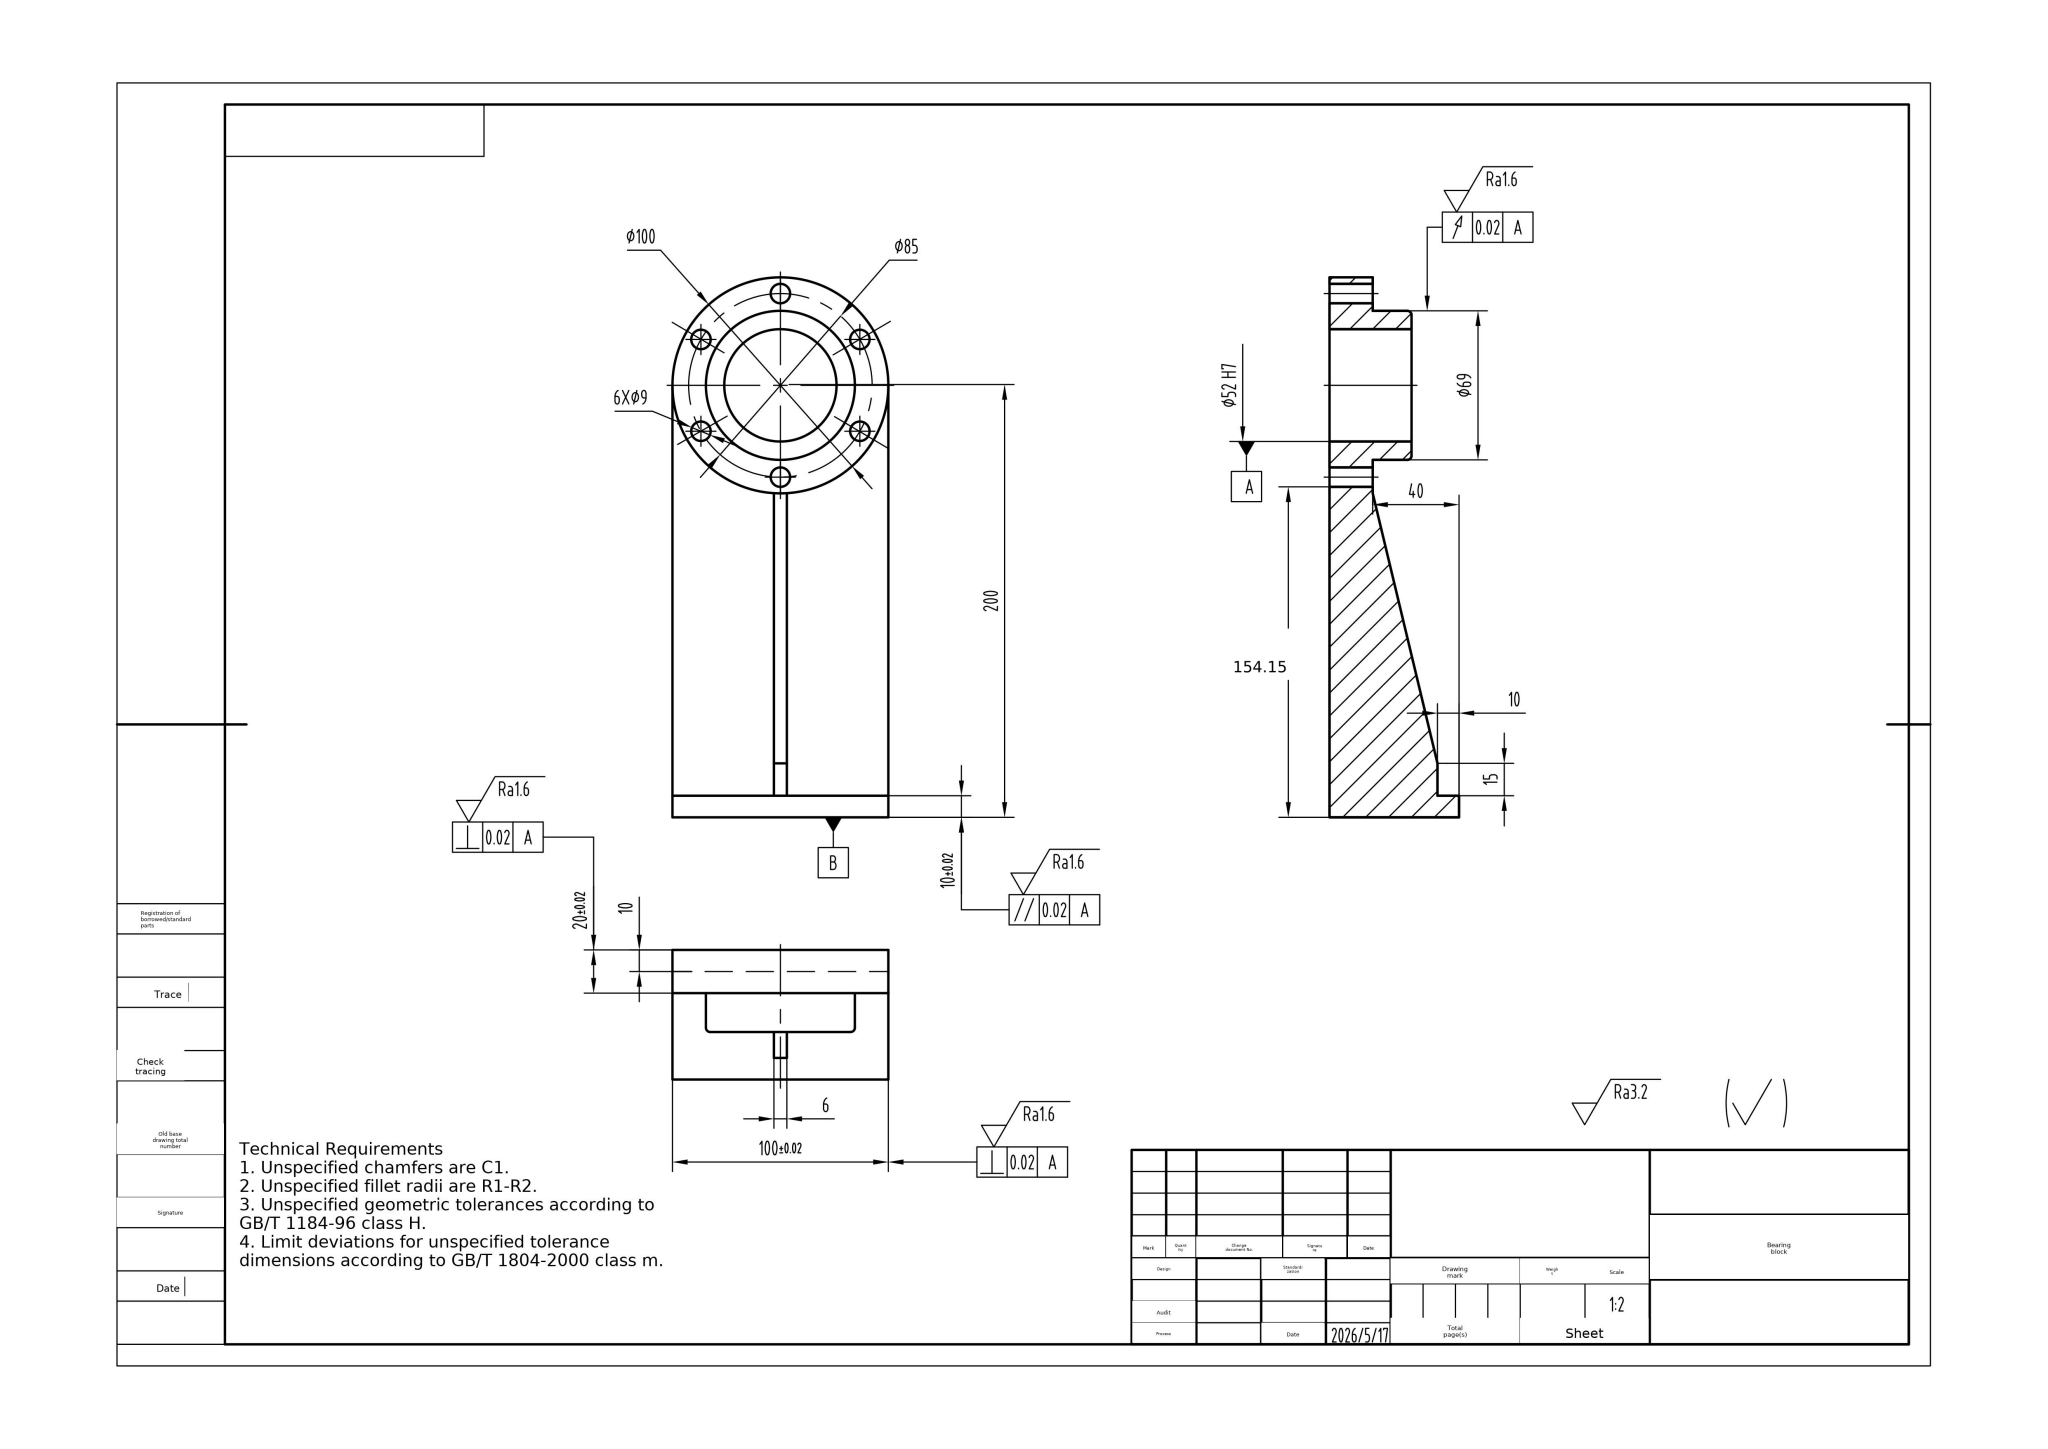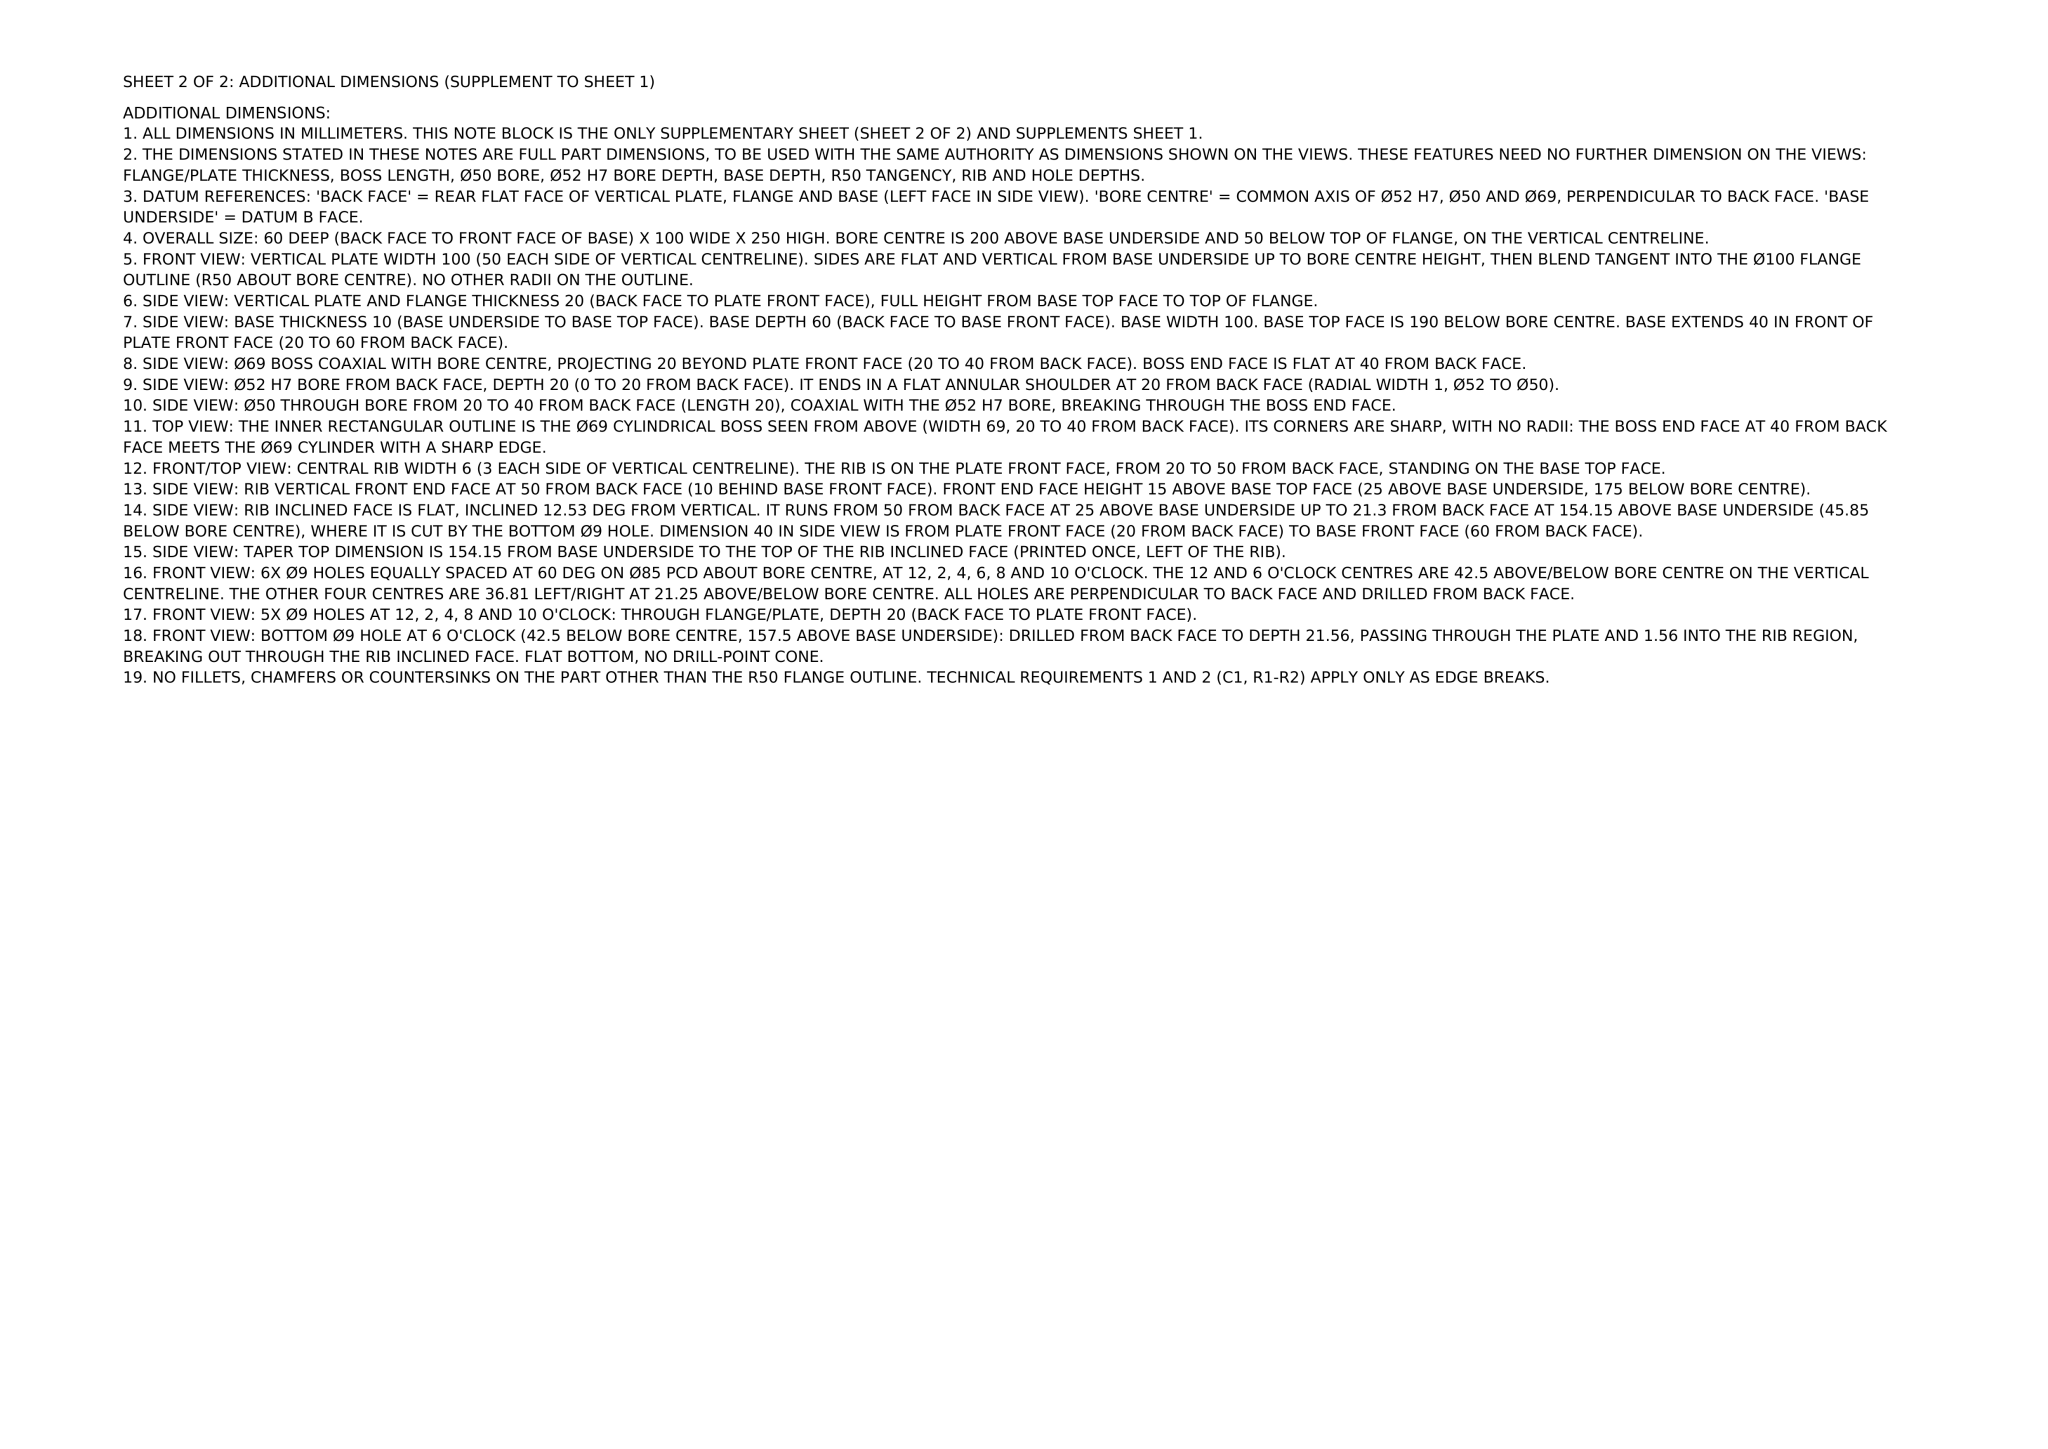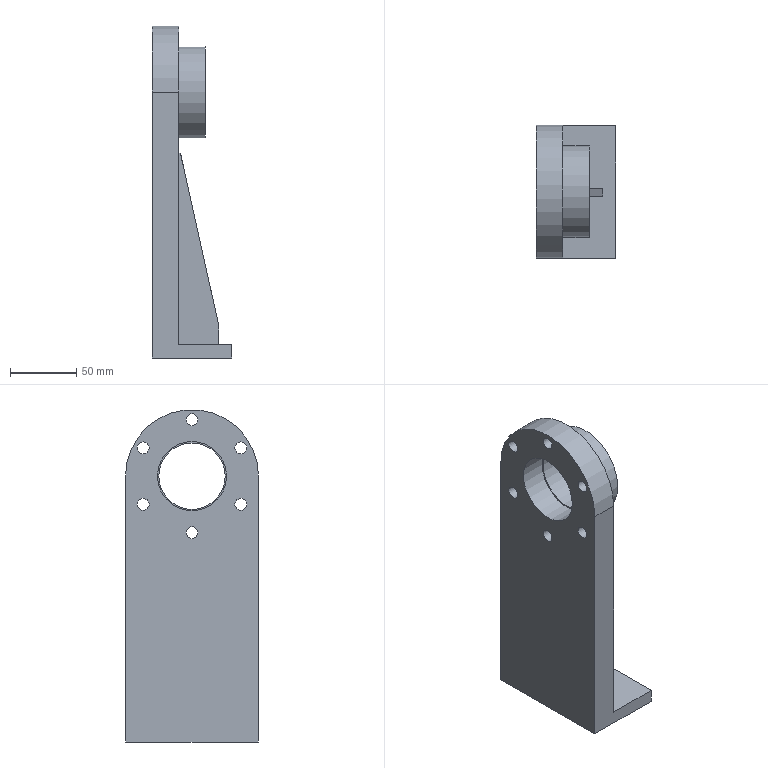Part | NX | mm | 1 solid | 23 faces | box 60 x 100 x 250 mm | volume 518768 mm3 | plane 13 | cylinder 10 | commonest cylinder face diameters 9 x6 100 x1 52 x1 69 x1 50 x1
STEP:
#1=CARTESIAN_POINT('',(0.,0.,0.));
#2=DIRECTION('',(0.,0.,1.));
#3=DIRECTION('',(1.,0.,0.));
#4=AXIS2_PLACEMENT_3D('',#1,#2,#3);
#5=(LENGTH_UNIT()NAMED_UNIT(*)SI_UNIT(.MILLI.,.METRE.));
#6=UNCERTAINTY_MEASURE_WITH_UNIT(LENGTH_MEASURE(0.00002),#5,'','');
#7=(NAMED_UNIT(*)PLANE_ANGLE_UNIT()SI_UNIT($,.RADIAN.));
#8=PLANE_ANGLE_MEASURE_WITH_UNIT(PLANE_ANGLE_MEASURE(0.01745),#7);
#9=DIMENSIONAL_EXPONENTS(0.,0.,0.,0.,0.,0.,0.);
#10=(CONVERSION_BASED_UNIT('',#8)NAMED_UNIT(#9)PLANE_ANGLE_UNIT());
#11=(NAMED_UNIT(*)SI_UNIT($,.STERADIAN.)SOLID_ANGLE_UNIT());
#12=(GEOMETRIC_REPRESENTATION_CONTEXT(3)GLOBAL_UNCERTAINTY_ASSIGNED_CONTEXT((#6))GLOBAL_UNIT_ASSIGNED_CONTEXT((#5,#10,#11))REPRESENTATION_CONTEXT('',''));
#13=SHAPE_REPRESENTATION('',(#4),#12);
#14=CARTESIAN_POINT('',(20.,-36.806,16.75));
#15=VERTEX_POINT('',#14);
#16=CARTESIAN_POINT('',(20.,-36.806,21.25));
#17=DIRECTION('',(1.,0.,0.));
#18=DIRECTION('',(0.,0.,-1.));
#19=AXIS2_PLACEMENT_3D('',#16,#17,#18);
#20=CIRCLE('',#19,4.5);
#21=EDGE_CURVE('',#15,#15,#20,.T.);
#22=ORIENTED_EDGE('',*,*,#21,.F.);
#23=EDGE_LOOP('',(#22));
#24=FACE_BOUND('',#23,.T.);
#25=CARTESIAN_POINT('',(20.,3.,-45.854));
#26=VERTEX_POINT('',#25);
#27=CARTESIAN_POINT('',(20.,-3.,-45.854));
#28=VERTEX_POINT('',#27);
#29=CARTESIAN_POINT('',(20.,0.,-42.5));
#30=DIRECTION('',(1.,0.,0.));
#31=DIRECTION('',(0.,0.,-1.));
#32=AXIS2_PLACEMENT_3D('',#29,#30,#31);
#33=CIRCLE('',#32,4.5);
#34=EDGE_CURVE('',#26,#28,#33,.T.);
#35=ORIENTED_EDGE('',*,*,#34,.F.);
#36=CARTESIAN_POINT('',(20.,3.,-190.));
#37=VERTEX_POINT('',#36);
#38=CARTESIAN_POINT('',(20.,3.,-40.));
#39=DIRECTION('',(0.,0.,-1.));
#40=VECTOR('',#39,1.);
#41=LINE('',#38,#40);
#42=EDGE_CURVE('',#26,#37,#41,.T.);
#43=ORIENTED_EDGE('',*,*,#42,.T.);
#44=CARTESIAN_POINT('',(20.,50.,-190.));
#45=VERTEX_POINT('',#44);
#46=CARTESIAN_POINT('',(20.,0.,-190.));
#47=DIRECTION('',(0.,1.,0.));
#48=VECTOR('',#47,1.);
#49=LINE('',#46,#48);
#50=EDGE_CURVE('',#37,#45,#49,.T.);
#51=ORIENTED_EDGE('',*,*,#50,.T.);
#52=CARTESIAN_POINT('',(20.,50.,0.));
#53=VERTEX_POINT('',#52);
#54=CARTESIAN_POINT('',(20.,50.,-200.));
#55=DIRECTION('',(0.,0.,1.));
#56=VECTOR('',#55,1.);
#57=LINE('',#54,#56);
#58=EDGE_CURVE('',#45,#53,#57,.T.);
#59=ORIENTED_EDGE('',*,*,#58,.T.);
#60=CARTESIAN_POINT('',(20.,-50.,0.));
#61=VERTEX_POINT('',#60);
#62=CARTESIAN_POINT('',(20.,0.,0.));
#63=DIRECTION('',(1.,0.,0.));
#64=DIRECTION('',(0.,1.,-0.));
#65=AXIS2_PLACEMENT_3D('',#62,#63,#64);
#66=CIRCLE('',#65,50.);
#67=EDGE_CURVE('',#53,#61,#66,.T.);
#68=ORIENTED_EDGE('',*,*,#67,.T.);
#69=CARTESIAN_POINT('',(20.,-50.,-190.));
#70=VERTEX_POINT('',#69);
#71=CARTESIAN_POINT('',(20.,-50.,0.));
#72=DIRECTION('',(0.,0.,-1.));
#73=VECTOR('',#72,1.);
#74=LINE('',#71,#73);
#75=EDGE_CURVE('',#61,#70,#74,.T.);
#76=ORIENTED_EDGE('',*,*,#75,.T.);
#77=CARTESIAN_POINT('',(20.,-3.,-190.));
#78=VERTEX_POINT('',#77);
#79=CARTESIAN_POINT('',(20.,0.,-190.));
#80=DIRECTION('',(0.,1.,0.));
#81=VECTOR('',#80,1.);
#82=LINE('',#79,#81);
#83=EDGE_CURVE('',#70,#78,#82,.T.);
#84=ORIENTED_EDGE('',*,*,#83,.T.);
#85=CARTESIAN_POINT('',(20.,-3.,-40.));
#86=DIRECTION('',(0.,0.,-1.));
#87=VECTOR('',#86,1.);
#88=LINE('',#85,#87);
#89=EDGE_CURVE('',#28,#78,#88,.T.);
#90=ORIENTED_EDGE('',*,*,#89,.F.);
#91=EDGE_LOOP('',(#35,#43,#51,#59,#68,#76,#84,#90));
#92=FACE_BOUND('',#91,.T.);
#93=CARTESIAN_POINT('',(20.,0.,38.));
#94=VERTEX_POINT('',#93);
#95=CARTESIAN_POINT('',(20.,0.,42.5));
#96=DIRECTION('',(1.,0.,0.));
#97=DIRECTION('',(0.,0.,-1.));
#98=AXIS2_PLACEMENT_3D('',#95,#96,#97);
#99=CIRCLE('',#98,4.5);
#100=EDGE_CURVE('',#94,#94,#99,.T.);
#101=ORIENTED_EDGE('',*,*,#100,.F.);
#102=EDGE_LOOP('',(#101));
#103=FACE_BOUND('',#102,.T.);
#104=CARTESIAN_POINT('',(20.,36.806,-25.75));
#105=VERTEX_POINT('',#104);
#106=CARTESIAN_POINT('',(20.,36.806,-21.25));
#107=DIRECTION('',(1.,0.,0.));
#108=DIRECTION('',(0.,0.,-1.));
#109=AXIS2_PLACEMENT_3D('',#106,#107,#108);
#110=CIRCLE('',#109,4.5);
#111=EDGE_CURVE('',#105,#105,#110,.T.);
#112=ORIENTED_EDGE('',*,*,#111,.F.);
#113=EDGE_LOOP('',(#112));
#114=FACE_BOUND('',#113,.T.);
#115=CARTESIAN_POINT('',(20.,-36.806,-25.75));
#116=VERTEX_POINT('',#115);
#117=CARTESIAN_POINT('',(20.,-36.806,-21.25));
#118=DIRECTION('',(1.,0.,0.));
#119=DIRECTION('',(0.,0.,-1.));
#120=AXIS2_PLACEMENT_3D('',#117,#118,#119);
#121=CIRCLE('',#120,4.5);
#122=EDGE_CURVE('',#116,#116,#121,.T.);
#123=ORIENTED_EDGE('',*,*,#122,.F.);
#124=EDGE_LOOP('',(#123));
#125=FACE_BOUND('',#124,.T.);
#126=CARTESIAN_POINT('',(20.,36.806,16.75));
#127=VERTEX_POINT('',#126);
#128=CARTESIAN_POINT('',(20.,36.806,21.25));
#129=DIRECTION('',(1.,0.,0.));
#130=DIRECTION('',(0.,0.,-1.));
#131=AXIS2_PLACEMENT_3D('',#128,#129,#130);
#132=CIRCLE('',#131,4.5);
#133=EDGE_CURVE('',#127,#127,#132,.T.);
#134=ORIENTED_EDGE('',*,*,#133,.F.);
#135=EDGE_LOOP('',(#134));
#136=FACE_BOUND('',#135,.T.);
#137=CARTESIAN_POINT('',(20.,34.5,-0.));
#138=VERTEX_POINT('',#137);
#139=CARTESIAN_POINT('',(20.,0.,0.));
#140=DIRECTION('',(1.,0.,0.));
#141=DIRECTION('',(0.,1.,-0.));
#142=AXIS2_PLACEMENT_3D('',#139,#140,#141);
#143=CIRCLE('',#142,34.5);
#144=EDGE_CURVE('',#138,#138,#143,.T.);
#145=ORIENTED_EDGE('',*,*,#144,.F.);
#146=EDGE_LOOP('',(#145));
#147=FACE_BOUND('',#146,.T.);
#148=CARTESIAN_POINT('',(20.,0.,0.));
#149=DIRECTION('',(1.,0.,0.));
#150=DIRECTION('',(0.,0.,-1.));
#151=AXIS2_PLACEMENT_3D('',#148,#149,#150);
#152=PLANE('',#151);
#153=ADVANCED_FACE('',(#24,#92,#103,#114,#125,#136,#147),#152,.T.);
#154=CARTESIAN_POINT('',(60.,-50.,-200.));
#155=VERTEX_POINT('',#154);
#156=CARTESIAN_POINT('',(0.,-50.,-200.));
#157=VERTEX_POINT('',#156);
#158=CARTESIAN_POINT('',(20.,-50.,-200.));
#159=DIRECTION('',(-1.,0.,0.));
#160=VECTOR('',#159,1.);
#161=LINE('',#158,#160);
#162=EDGE_CURVE('',#155,#157,#161,.T.);
#163=ORIENTED_EDGE('',*,*,#162,.F.);
#164=CARTESIAN_POINT('',(60.,-50.,-190.));
#165=VERTEX_POINT('',#164);
#166=CARTESIAN_POINT('',(60.,-50.,-190.));
#167=DIRECTION('',(0.,0.,-1.));
#168=VECTOR('',#167,1.);
#169=LINE('',#166,#168);
#170=EDGE_CURVE('',#165,#155,#169,.T.);
#171=ORIENTED_EDGE('',*,*,#170,.F.);
#172=CARTESIAN_POINT('',(60.,-50.,-190.));
#173=DIRECTION('',(-1.,0.,0.));
#174=VECTOR('',#173,1.);
#175=LINE('',#172,#174);
#176=EDGE_CURVE('',#165,#70,#175,.T.);
#177=ORIENTED_EDGE('',*,*,#176,.T.);
#178=ORIENTED_EDGE('',*,*,#75,.F.);
#179=CARTESIAN_POINT('',(0.,-50.,0.));
#180=VERTEX_POINT('',#179);
#181=CARTESIAN_POINT('',(20.,-50.,0.));
#182=DIRECTION('',(-1.,0.,0.));
#183=VECTOR('',#182,1.);
#184=LINE('',#181,#183);
#185=EDGE_CURVE('',#61,#180,#184,.T.);
#186=ORIENTED_EDGE('',*,*,#185,.T.);
#187=CARTESIAN_POINT('',(0.,-50.,0.));
#188=DIRECTION('',(0.,0.,-1.));
#189=VECTOR('',#188,1.);
#190=LINE('',#187,#189);
#191=EDGE_CURVE('',#180,#157,#190,.T.);
#192=ORIENTED_EDGE('',*,*,#191,.T.);
#193=EDGE_LOOP('',(#163,#171,#177,#178,#186,#192));
#194=FACE_OUTER_BOUND('',#193,.T.);
#195=CARTESIAN_POINT('',(20.,-50.,0.));
#196=DIRECTION('',(0.,1.,0.));
#197=DIRECTION('',(0.,-0.,1.));
#198=AXIS2_PLACEMENT_3D('',#195,#196,#197);
#199=PLANE('',#198);
#200=ADVANCED_FACE('',(#194),#199,.F.);
#201=CARTESIAN_POINT('',(0.,50.,-200.));
#202=VERTEX_POINT('',#201);
#203=CARTESIAN_POINT('',(0.,-50.,-200.));
#204=DIRECTION('',(0.,1.,0.));
#205=VECTOR('',#204,1.);
#206=LINE('',#203,#205);
#207=EDGE_CURVE('',#157,#202,#206,.T.);
#208=ORIENTED_EDGE('',*,*,#207,.T.);
#209=CARTESIAN_POINT('',(60.,50.,-200.));
#210=VERTEX_POINT('',#209);
#211=CARTESIAN_POINT('',(20.,50.,-200.));
#212=DIRECTION('',(-1.,0.,0.));
#213=VECTOR('',#212,1.);
#214=LINE('',#211,#213);
#215=EDGE_CURVE('',#210,#202,#214,.T.);
#216=ORIENTED_EDGE('',*,*,#215,.F.);
#217=CARTESIAN_POINT('',(60.,50.,-200.));
#218=DIRECTION('',(-0.,-1.,0.));
#219=VECTOR('',#218,1.);
#220=LINE('',#217,#219);
#221=EDGE_CURVE('',#210,#155,#220,.T.);
#222=ORIENTED_EDGE('',*,*,#221,.T.);
#223=ORIENTED_EDGE('',*,*,#162,.T.);
#224=EDGE_LOOP('',(#208,#216,#222,#223));
#225=FACE_OUTER_BOUND('',#224,.T.);
#226=CARTESIAN_POINT('',(20.,-50.,-200.));
#227=DIRECTION('',(0.,0.,1.));
#228=DIRECTION('',(1.,0.,0.));
#229=AXIS2_PLACEMENT_3D('',#226,#227,#228);
#230=PLANE('',#229);
#231=ADVANCED_FACE('',(#225),#230,.F.);
#232=CARTESIAN_POINT('',(0.,50.,0.));
#233=VERTEX_POINT('',#232);
#234=CARTESIAN_POINT('',(0.,50.,-200.));
#235=DIRECTION('',(0.,0.,1.));
#236=VECTOR('',#235,1.);
#237=LINE('',#234,#236);
#238=EDGE_CURVE('',#202,#233,#237,.T.);
#239=ORIENTED_EDGE('',*,*,#238,.T.);
#240=CARTESIAN_POINT('',(20.,50.,0.));
#241=DIRECTION('',(-1.,0.,0.));
#242=VECTOR('',#241,1.);
#243=LINE('',#240,#242);
#244=EDGE_CURVE('',#53,#233,#243,.T.);
#245=ORIENTED_EDGE('',*,*,#244,.F.);
#246=ORIENTED_EDGE('',*,*,#58,.F.);
#247=CARTESIAN_POINT('',(60.,50.,-190.));
#248=VERTEX_POINT('',#247);
#249=CARTESIAN_POINT('',(0.,50.,-190.));
#250=DIRECTION('',(1.,-0.,0.));
#251=VECTOR('',#250,1.);
#252=LINE('',#249,#251);
#253=EDGE_CURVE('',#45,#248,#252,.T.);
#254=ORIENTED_EDGE('',*,*,#253,.T.);
#255=CARTESIAN_POINT('',(60.,50.,-190.));
#256=DIRECTION('',(0.,0.,-1.));
#257=VECTOR('',#256,1.);
#258=LINE('',#255,#257);
#259=EDGE_CURVE('',#248,#210,#258,.T.);
#260=ORIENTED_EDGE('',*,*,#259,.T.);
#261=ORIENTED_EDGE('',*,*,#215,.T.);
#262=EDGE_LOOP('',(#239,#245,#246,#254,#260,#261));
#263=FACE_OUTER_BOUND('',#262,.T.);
#264=CARTESIAN_POINT('',(20.,50.,-200.));
#265=DIRECTION('',(0.,-1.,0.));
#266=DIRECTION('',(0.,0.,-1.));
#267=AXIS2_PLACEMENT_3D('',#264,#265,#266);
#268=PLANE('',#267);
#269=ADVANCED_FACE('',(#263),#268,.F.);
#270=CARTESIAN_POINT('',(0.,0.,0.));
#271=DIRECTION('',(1.,0.,0.));
#272=DIRECTION('',(0.,1.,-0.));
#273=AXIS2_PLACEMENT_3D('',#270,#271,#272);
#274=CIRCLE('',#273,50.);
#275=EDGE_CURVE('',#233,#180,#274,.T.);
#276=ORIENTED_EDGE('',*,*,#275,.T.);
#277=ORIENTED_EDGE('',*,*,#185,.F.);
#278=ORIENTED_EDGE('',*,*,#67,.F.);
#279=ORIENTED_EDGE('',*,*,#244,.T.);
#280=EDGE_LOOP('',(#276,#277,#278,#279));
#281=FACE_OUTER_BOUND('',#280,.T.);
#282=CARTESIAN_POINT('',(20.,0.,0.));
#283=DIRECTION('',(-1.,0.,0.));
#284=DIRECTION('',(0.,0.,1.));
#285=AXIS2_PLACEMENT_3D('',#282,#283,#284);
#286=CYLINDRICAL_SURFACE('',#285,50.);
#287=ADVANCED_FACE('',(#281),#286,.T.);
#288=CARTESIAN_POINT('',(20.,26.,-0.));
#289=VERTEX_POINT('',#288);
#290=CARTESIAN_POINT('',(20.,0.,0.));
#291=DIRECTION('',(1.,0.,0.));
#292=DIRECTION('',(0.,1.,-0.));
#293=AXIS2_PLACEMENT_3D('',#290,#291,#292);
#294=CIRCLE('',#293,26.);
#295=EDGE_CURVE('',#289,#289,#294,.T.);
#296=ORIENTED_EDGE('',*,*,#295,.T.);
#297=EDGE_LOOP('',(#296));
#298=FACE_BOUND('',#297,.T.);
#299=CARTESIAN_POINT('',(0.,26.,-0.));
#300=VERTEX_POINT('',#299);
#301=CARTESIAN_POINT('',(0.,0.,0.));
#302=DIRECTION('',(1.,0.,0.));
#303=DIRECTION('',(0.,1.,-0.));
#304=AXIS2_PLACEMENT_3D('',#301,#302,#303);
#305=CIRCLE('',#304,26.);
#306=EDGE_CURVE('',#300,#300,#305,.T.);
#307=ORIENTED_EDGE('',*,*,#306,.F.);
#308=EDGE_LOOP('',(#307));
#309=FACE_BOUND('',#308,.T.);
#310=CARTESIAN_POINT('',(20.,0.,0.));
#311=DIRECTION('',(-1.,0.,0.));
#312=DIRECTION('',(0.,0.,1.));
#313=AXIS2_PLACEMENT_3D('',#310,#311,#312);
#314=CYLINDRICAL_SURFACE('',#313,26.);
#315=ADVANCED_FACE('',(#298,#309),#314,.F.);
#316=CARTESIAN_POINT('',(0.,-36.806,16.75));
#317=VERTEX_POINT('',#316);
#318=CARTESIAN_POINT('',(0.,-36.806,21.25));
#319=DIRECTION('',(1.,0.,0.));
#320=DIRECTION('',(0.,0.,-1.));
#321=AXIS2_PLACEMENT_3D('',#318,#319,#320);
#322=CIRCLE('',#321,4.5);
#323=EDGE_CURVE('',#317,#317,#322,.T.);
#324=ORIENTED_EDGE('',*,*,#323,.T.);
#325=EDGE_LOOP('',(#324));
#326=FACE_BOUND('',#325,.T.);
#327=CARTESIAN_POINT('',(0.,0.,-47.));
#328=VERTEX_POINT('',#327);
#329=CARTESIAN_POINT('',(0.,0.,-42.5));
#330=DIRECTION('',(1.,0.,0.));
#331=DIRECTION('',(0.,0.,-1.));
#332=AXIS2_PLACEMENT_3D('',#329,#330,#331);
#333=CIRCLE('',#332,4.5);
#334=EDGE_CURVE('',#328,#328,#333,.T.);
#335=ORIENTED_EDGE('',*,*,#334,.T.);
#336=EDGE_LOOP('',(#335));
#337=FACE_BOUND('',#336,.T.);
#338=CARTESIAN_POINT('',(0.,0.,38.));
#339=VERTEX_POINT('',#338);
#340=CARTESIAN_POINT('',(0.,0.,42.5));
#341=DIRECTION('',(1.,0.,0.));
#342=DIRECTION('',(0.,0.,-1.));
#343=AXIS2_PLACEMENT_3D('',#340,#341,#342);
#344=CIRCLE('',#343,4.5);
#345=EDGE_CURVE('',#339,#339,#344,.T.);
#346=ORIENTED_EDGE('',*,*,#345,.T.);
#347=EDGE_LOOP('',(#346));
#348=FACE_BOUND('',#347,.T.);
#349=CARTESIAN_POINT('',(0.,36.806,-25.75));
#350=VERTEX_POINT('',#349);
#351=CARTESIAN_POINT('',(0.,36.806,-21.25));
#352=DIRECTION('',(1.,0.,0.));
#353=DIRECTION('',(0.,0.,-1.));
#354=AXIS2_PLACEMENT_3D('',#351,#352,#353);
#355=CIRCLE('',#354,4.5);
#356=EDGE_CURVE('',#350,#350,#355,.T.);
#357=ORIENTED_EDGE('',*,*,#356,.T.);
#358=EDGE_LOOP('',(#357));
#359=FACE_BOUND('',#358,.T.);
#360=CARTESIAN_POINT('',(0.,-36.806,-25.75));
#361=VERTEX_POINT('',#360);
#362=CARTESIAN_POINT('',(0.,-36.806,-21.25));
#363=DIRECTION('',(1.,0.,0.));
#364=DIRECTION('',(0.,0.,-1.));
#365=AXIS2_PLACEMENT_3D('',#362,#363,#364);
#366=CIRCLE('',#365,4.5);
#367=EDGE_CURVE('',#361,#361,#366,.T.);
#368=ORIENTED_EDGE('',*,*,#367,.T.);
#369=EDGE_LOOP('',(#368));
#370=FACE_BOUND('',#369,.T.);
#371=CARTESIAN_POINT('',(0.,36.806,16.75));
#372=VERTEX_POINT('',#371);
#373=CARTESIAN_POINT('',(0.,36.806,21.25));
#374=DIRECTION('',(1.,0.,0.));
#375=DIRECTION('',(0.,0.,-1.));
#376=AXIS2_PLACEMENT_3D('',#373,#374,#375);
#377=CIRCLE('',#376,4.5);
#378=EDGE_CURVE('',#372,#372,#377,.T.);
#379=ORIENTED_EDGE('',*,*,#378,.T.);
#380=EDGE_LOOP('',(#379));
#381=FACE_BOUND('',#380,.T.);
#382=ORIENTED_EDGE('',*,*,#207,.F.);
#383=ORIENTED_EDGE('',*,*,#191,.F.);
#384=ORIENTED_EDGE('',*,*,#275,.F.);
#385=ORIENTED_EDGE('',*,*,#238,.F.);
#386=EDGE_LOOP('',(#382,#383,#384,#385));
#387=FACE_BOUND('',#386,.T.);
#388=ORIENTED_EDGE('',*,*,#306,.T.);
#389=EDGE_LOOP('',(#388));
#390=FACE_BOUND('',#389,.T.);
#391=CARTESIAN_POINT('',(0.,0.,0.));
#392=DIRECTION('',(1.,0.,0.));
#393=DIRECTION('',(0.,0.,-1.));
#394=AXIS2_PLACEMENT_3D('',#391,#392,#393);
#395=PLANE('',#394);
#396=ADVANCED_FACE('',(#326,#337,#348,#359,#370,#381,#387,#390),#395,.F.);
#397=CARTESIAN_POINT('',(40.,34.5,-0.));
#398=VERTEX_POINT('',#397);
#399=CARTESIAN_POINT('',(40.,0.,0.));
#400=DIRECTION('',(1.,0.,0.));
#401=DIRECTION('',(0.,1.,-0.));
#402=AXIS2_PLACEMENT_3D('',#399,#400,#401);
#403=CIRCLE('',#402,34.5);
#404=EDGE_CURVE('',#398,#398,#403,.T.);
#405=ORIENTED_EDGE('',*,*,#404,.F.);
#406=EDGE_LOOP('',(#405));
#407=FACE_BOUND('',#406,.T.);
#408=ORIENTED_EDGE('',*,*,#144,.T.);
#409=EDGE_LOOP('',(#408));
#410=FACE_BOUND('',#409,.T.);
#411=CARTESIAN_POINT('',(40.,0.,0.));
#412=DIRECTION('',(-1.,0.,0.));
#413=DIRECTION('',(0.,0.,1.));
#414=AXIS2_PLACEMENT_3D('',#411,#412,#413);
#415=CYLINDRICAL_SURFACE('',#414,34.5);
#416=ADVANCED_FACE('',(#407,#410),#415,.T.);
#417=CARTESIAN_POINT('',(40.,25.,-0.));
#418=VERTEX_POINT('',#417);
#419=CARTESIAN_POINT('',(40.,0.,0.));
#420=DIRECTION('',(1.,0.,0.));
#421=DIRECTION('',(0.,1.,-0.));
#422=AXIS2_PLACEMENT_3D('',#419,#420,#421);
#423=CIRCLE('',#422,25.);
#424=EDGE_CURVE('',#418,#418,#423,.T.);
#425=ORIENTED_EDGE('',*,*,#424,.T.);
#426=EDGE_LOOP('',(#425));
#427=FACE_BOUND('',#426,.T.);
#428=CARTESIAN_POINT('',(20.,25.,-0.));
#429=VERTEX_POINT('',#428);
#430=CARTESIAN_POINT('',(20.,0.,0.));
#431=DIRECTION('',(1.,0.,0.));
#432=DIRECTION('',(0.,1.,-0.));
#433=AXIS2_PLACEMENT_3D('',#430,#431,#432);
#434=CIRCLE('',#433,25.);
#435=EDGE_CURVE('',#429,#429,#434,.T.);
#436=ORIENTED_EDGE('',*,*,#435,.F.);
#437=EDGE_LOOP('',(#436));
#438=FACE_BOUND('',#437,.T.);
#439=CARTESIAN_POINT('',(40.,0.,0.));
#440=DIRECTION('',(-1.,0.,0.));
#441=DIRECTION('',(0.,0.,1.));
#442=AXIS2_PLACEMENT_3D('',#439,#440,#441);
#443=CYLINDRICAL_SURFACE('',#442,25.);
#444=ADVANCED_FACE('',(#427,#438),#443,.F.);
#445=ORIENTED_EDGE('',*,*,#404,.T.);
#446=EDGE_LOOP('',(#445));
#447=FACE_BOUND('',#446,.T.);
#448=ORIENTED_EDGE('',*,*,#424,.F.);
#449=EDGE_LOOP('',(#448));
#450=FACE_BOUND('',#449,.T.);
#451=CARTESIAN_POINT('',(40.,0.,0.));
#452=DIRECTION('',(1.,0.,0.));
#453=DIRECTION('',(0.,0.,-1.));
#454=AXIS2_PLACEMENT_3D('',#451,#452,#453);
#455=PLANE('',#454);
#456=ADVANCED_FACE('',(#447,#450),#455,.T.);
#457=ORIENTED_EDGE('',*,*,#295,.F.);
#458=EDGE_LOOP('',(#457));
#459=FACE_BOUND('',#458,.T.);
#460=ORIENTED_EDGE('',*,*,#435,.T.);
#461=EDGE_LOOP('',(#460));
#462=FACE_BOUND('',#461,.T.);
#463=CARTESIAN_POINT('',(20.,0.,0.));
#464=DIRECTION('',(1.,0.,0.));
#465=DIRECTION('',(0.,0.,-1.));
#466=AXIS2_PLACEMENT_3D('',#463,#464,#465);
#467=PLANE('',#466);
#468=ADVANCED_FACE('',(#459,#462),#467,.F.);
#469=ORIENTED_EDGE('',*,*,#221,.F.);
#470=ORIENTED_EDGE('',*,*,#259,.F.);
#471=CARTESIAN_POINT('',(60.,50.,-190.));
#472=DIRECTION('',(-0.,-1.,0.));
#473=VECTOR('',#472,1.);
#474=LINE('',#471,#473);
#475=EDGE_CURVE('',#248,#165,#474,.T.);
#476=ORIENTED_EDGE('',*,*,#475,.T.);
#477=ORIENTED_EDGE('',*,*,#170,.T.);
#478=EDGE_LOOP('',(#469,#470,#476,#477));
#479=FACE_OUTER_BOUND('',#478,.T.);
#480=CARTESIAN_POINT('',(60.,50.,-190.));
#481=DIRECTION('',(1.,-0.,0.));
#482=DIRECTION('',(0.,1.,0.));
#483=AXIS2_PLACEMENT_3D('',#480,#481,#482);
#484=PLANE('',#483);
#485=ADVANCED_FACE('',(#479),#484,.T.);
#486=ORIENTED_EDGE('',*,*,#50,.F.);
#487=CARTESIAN_POINT('',(50.,3.,-190.));
#488=VERTEX_POINT('',#487);
#489=CARTESIAN_POINT('',(20.,3.,-190.));
#490=DIRECTION('',(1.,0.,-0.));
#491=VECTOR('',#490,1.);
#492=LINE('',#489,#491);
#493=EDGE_CURVE('',#37,#488,#492,.T.);
#494=ORIENTED_EDGE('',*,*,#493,.T.);
#495=CARTESIAN_POINT('',(50.,-3.,-190.));
#496=VERTEX_POINT('',#495);
#497=CARTESIAN_POINT('',(50.,-3.,-190.));
#498=DIRECTION('',(0.,1.,0.));
#499=VECTOR('',#498,1.);
#500=LINE('',#497,#499);
#501=EDGE_CURVE('',#496,#488,#500,.T.);
#502=ORIENTED_EDGE('',*,*,#501,.F.);
#503=CARTESIAN_POINT('',(20.,-3.,-190.));
#504=DIRECTION('',(1.,0.,-0.));
#505=VECTOR('',#504,1.);
#506=LINE('',#503,#505);
#507=EDGE_CURVE('',#78,#496,#506,.T.);
#508=ORIENTED_EDGE('',*,*,#507,.F.);
#509=ORIENTED_EDGE('',*,*,#83,.F.);
#510=ORIENTED_EDGE('',*,*,#176,.F.);
#511=ORIENTED_EDGE('',*,*,#475,.F.);
#512=ORIENTED_EDGE('',*,*,#253,.F.);
#513=EDGE_LOOP('',(#486,#494,#502,#508,#509,#510,#511,#512));
#514=FACE_OUTER_BOUND('',#513,.T.);
#515=CARTESIAN_POINT('',(0.,0.,-190.));
#516=DIRECTION('',(0.,0.,-1.));
#517=DIRECTION('',(-1.,0.,0.));
#518=AXIS2_PLACEMENT_3D('',#515,#516,#517);
#519=PLANE('',#518);
#520=ADVANCED_FACE('',(#514),#519,.F.);
#521=CARTESIAN_POINT('',(50.,3.,-175.));
#522=VERTEX_POINT('',#521);
#523=CARTESIAN_POINT('',(21.301,3.,-45.854));
#524=VERTEX_POINT('',#523);
#525=CARTESIAN_POINT('',(50.,3.,-175.));
#526=DIRECTION('',(-0.2169,0.,0.9762));
#527=VECTOR('',#526,1.);
#528=LINE('',#525,#527);
#529=EDGE_CURVE('',#522,#524,#528,.T.);
#530=ORIENTED_EDGE('',*,*,#529,.T.);
#531=CARTESIAN_POINT('',(21.301,-3.,-45.854));
#532=VERTEX_POINT('',#531);
#533=CARTESIAN_POINT('',(20.556,0.,-42.5));
#534=DIRECTION('',(-0.9762,0.,-0.2169));
#535=DIRECTION('',(0.2169,0.,-0.9762));
#536=AXIS2_PLACEMENT_3D('',#533,#534,#535);
#537=ELLIPSE('',#536,4.61,4.5);
#538=EDGE_CURVE('',#524,#532,#537,.T.);
#539=ORIENTED_EDGE('',*,*,#538,.T.);
#540=CARTESIAN_POINT('',(50.,-3.,-175.));
#541=VERTEX_POINT('',#540);
#542=CARTESIAN_POINT('',(50.,-3.,-175.));
#543=DIRECTION('',(-0.2169,0.,0.9762));
#544=VECTOR('',#543,1.);
#545=LINE('',#542,#544);
#546=EDGE_CURVE('',#541,#532,#545,.T.);
#547=ORIENTED_EDGE('',*,*,#546,.F.);
#548=CARTESIAN_POINT('',(50.,-3.,-175.));
#549=DIRECTION('',(0.,1.,0.));
#550=VECTOR('',#549,1.);
#551=LINE('',#548,#550);
#552=EDGE_CURVE('',#541,#522,#551,.T.);
#553=ORIENTED_EDGE('',*,*,#552,.T.);
#554=EDGE_LOOP('',(#530,#539,#547,#553));
#555=FACE_OUTER_BOUND('',#554,.T.);
#556=CARTESIAN_POINT('',(50.,-3.,-175.));
#557=DIRECTION('',(-0.9762,0.,-0.2169));
#558=DIRECTION('',(-0.2169,0.,0.9762));
#559=AXIS2_PLACEMENT_3D('',#556,#557,#558);
#560=PLANE('',#559);
#561=ADVANCED_FACE('',(#555),#560,.F.);
#562=CARTESIAN_POINT('',(50.,3.,-190.));
#563=DIRECTION('',(0.,0.,1.));
#564=VECTOR('',#563,1.);
#565=LINE('',#562,#564);
#566=EDGE_CURVE('',#488,#522,#565,.T.);
#567=ORIENTED_EDGE('',*,*,#566,.T.);
#568=ORIENTED_EDGE('',*,*,#552,.F.);
#569=CARTESIAN_POINT('',(50.,-3.,-190.));
#570=DIRECTION('',(0.,0.,1.));
#571=VECTOR('',#570,1.);
#572=LINE('',#569,#571);
#573=EDGE_CURVE('',#496,#541,#572,.T.);
#574=ORIENTED_EDGE('',*,*,#573,.F.);
#575=ORIENTED_EDGE('',*,*,#501,.T.);
#576=EDGE_LOOP('',(#567,#568,#574,#575));
#577=FACE_OUTER_BOUND('',#576,.T.);
#578=CARTESIAN_POINT('',(50.,-3.,-190.));
#579=DIRECTION('',(-1.,0.,0.));
#580=DIRECTION('',(0.,0.,1.));
#581=AXIS2_PLACEMENT_3D('',#578,#579,#580);
#582=PLANE('',#581);
#583=ADVANCED_FACE('',(#577),#582,.F.);
#584=ORIENTED_EDGE('',*,*,#546,.T.);
#585=CARTESIAN_POINT('',(-30.,-3.,-45.854));
#586=DIRECTION('',(-1.,0.,0.));
#587=VECTOR('',#586,1.);
#588=LINE('',#585,#587);
#589=EDGE_CURVE('',#532,#28,#588,.T.);
#590=ORIENTED_EDGE('',*,*,#589,.T.);
#591=ORIENTED_EDGE('',*,*,#89,.T.);
#592=ORIENTED_EDGE('',*,*,#507,.T.);
#593=ORIENTED_EDGE('',*,*,#573,.T.);
#594=EDGE_LOOP('',(#584,#590,#591,#592,#593));
#595=FACE_OUTER_BOUND('',#594,.T.);
#596=CARTESIAN_POINT('',(0.,-3.,0.));
#597=DIRECTION('',(0.,1.,0.));
#598=DIRECTION('',(0.,0.,1.));
#599=AXIS2_PLACEMENT_3D('',#596,#597,#598);
#600=PLANE('',#599);
#601=ADVANCED_FACE('',(#595),#600,.F.);
#602=CARTESIAN_POINT('',(-30.,3.,-45.854));
#603=DIRECTION('',(-1.,0.,0.));
#604=VECTOR('',#603,1.);
#605=LINE('',#602,#604);
#606=EDGE_CURVE('',#524,#26,#605,.T.);
#607=ORIENTED_EDGE('',*,*,#606,.F.);
#608=ORIENTED_EDGE('',*,*,#529,.F.);
#609=ORIENTED_EDGE('',*,*,#566,.F.);
#610=ORIENTED_EDGE('',*,*,#493,.F.);
#611=ORIENTED_EDGE('',*,*,#42,.F.);
#612=EDGE_LOOP('',(#607,#608,#609,#610,#611));
#613=FACE_OUTER_BOUND('',#612,.T.);
#614=CARTESIAN_POINT('',(0.,3.,0.));
#615=DIRECTION('',(0.,1.,0.));
#616=DIRECTION('',(0.,0.,1.));
#617=AXIS2_PLACEMENT_3D('',#614,#615,#616);
#618=PLANE('',#617);
#619=ADVANCED_FACE('',(#613),#618,.T.);
#620=ORIENTED_EDGE('',*,*,#538,.F.);
#621=ORIENTED_EDGE('',*,*,#606,.T.);
#622=ORIENTED_EDGE('',*,*,#34,.T.);
#623=ORIENTED_EDGE('',*,*,#589,.F.);
#624=EDGE_LOOP('',(#620,#621,#622,#623));
#625=FACE_BOUND('',#624,.T.);
#626=ORIENTED_EDGE('',*,*,#334,.F.);
#627=EDGE_LOOP('',(#626));
#628=FACE_BOUND('',#627,.T.);
#629=CARTESIAN_POINT('',(-30.,0.,-42.5));
#630=DIRECTION('',(1.,0.,0.));
#631=DIRECTION('',(0.,0.,-1.));
#632=AXIS2_PLACEMENT_3D('',#629,#630,#631);
#633=CYLINDRICAL_SURFACE('',#632,4.5);
#634=ADVANCED_FACE('',(#625,#628),#633,.F.);
#635=ORIENTED_EDGE('',*,*,#133,.T.);
#636=EDGE_LOOP('',(#635));
#637=FACE_BOUND('',#636,.T.);
#638=ORIENTED_EDGE('',*,*,#378,.F.);
#639=EDGE_LOOP('',(#638));
#640=FACE_BOUND('',#639,.T.);
#641=CARTESIAN_POINT('',(-30.,36.806,21.25));
#642=DIRECTION('',(1.,0.,0.));
#643=DIRECTION('',(0.,0.,-1.));
#644=AXIS2_PLACEMENT_3D('',#641,#642,#643);
#645=CYLINDRICAL_SURFACE('',#644,4.5);
#646=ADVANCED_FACE('',(#637,#640),#645,.F.);
#647=ORIENTED_EDGE('',*,*,#122,.T.);
#648=EDGE_LOOP('',(#647));
#649=FACE_BOUND('',#648,.T.);
#650=ORIENTED_EDGE('',*,*,#367,.F.);
#651=EDGE_LOOP('',(#650));
#652=FACE_BOUND('',#651,.T.);
#653=CARTESIAN_POINT('',(-30.,-36.806,-21.25));
#654=DIRECTION('',(1.,0.,0.));
#655=DIRECTION('',(0.,0.,-1.));
#656=AXIS2_PLACEMENT_3D('',#653,#654,#655);
#657=CYLINDRICAL_SURFACE('',#656,4.5);
#658=ADVANCED_FACE('',(#649,#652),#657,.F.);
#659=ORIENTED_EDGE('',*,*,#111,.T.);
#660=EDGE_LOOP('',(#659));
#661=FACE_BOUND('',#660,.T.);
#662=ORIENTED_EDGE('',*,*,#356,.F.);
#663=EDGE_LOOP('',(#662));
#664=FACE_BOUND('',#663,.T.);
#665=CARTESIAN_POINT('',(-30.,36.806,-21.25));
#666=DIRECTION('',(1.,0.,0.));
#667=DIRECTION('',(0.,0.,-1.));
#668=AXIS2_PLACEMENT_3D('',#665,#666,#667);
#669=CYLINDRICAL_SURFACE('',#668,4.5);
#670=ADVANCED_FACE('',(#661,#664),#669,.F.);
#671=ORIENTED_EDGE('',*,*,#100,.T.);
#672=EDGE_LOOP('',(#671));
#673=FACE_BOUND('',#672,.T.);
#674=ORIENTED_EDGE('',*,*,#345,.F.);
#675=EDGE_LOOP('',(#674));
#676=FACE_BOUND('',#675,.T.);
#677=CARTESIAN_POINT('',(-30.,0.,42.5));
#678=DIRECTION('',(1.,0.,0.));
#679=DIRECTION('',(0.,0.,-1.));
#680=AXIS2_PLACEMENT_3D('',#677,#678,#679);
#681=CYLINDRICAL_SURFACE('',#680,4.5);
#682=ADVANCED_FACE('',(#673,#676),#681,.F.);
#683=ORIENTED_EDGE('',*,*,#21,.T.);
#684=EDGE_LOOP('',(#683));
#685=FACE_BOUND('',#684,.T.);
#686=ORIENTED_EDGE('',*,*,#323,.F.);
#687=EDGE_LOOP('',(#686));
#688=FACE_BOUND('',#687,.T.);
#689=CARTESIAN_POINT('',(-30.,-36.806,21.25));
#690=DIRECTION('',(1.,0.,0.));
#691=DIRECTION('',(0.,0.,-1.));
#692=AXIS2_PLACEMENT_3D('',#689,#690,#691);
#693=CYLINDRICAL_SURFACE('',#692,4.5);
#694=ADVANCED_FACE('',(#685,#688),#693,.F.);
#695=CLOSED_SHELL('',(#153,#200,#231,#269,#287,#315,#396,#416,#444,#456,#468,#485,#520,#561,#583,#601,#619,#634,#646,#658,#670,#682,#694));
#696=MANIFOLD_SOLID_BREP('',#695);
#697=ADVANCED_BREP_SHAPE_REPRESENTATION('',(#696),#12);
#698=SHAPE_REPRESENTATION_RELATIONSHIP('','',#13,#697);
#699=PRESENTATION_LAYER_ASSIGNMENT('','',(#696));
#700=COLOUR_RGB('',1.,0.6,0.);
#701=FILL_AREA_STYLE_COLOUR('',#700);
#702=FILL_AREA_STYLE('',(#701));
#703=SURFACE_STYLE_FILL_AREA(#702);
#704=SURFACE_SIDE_STYLE('',(#703));
#705=SURFACE_STYLE_USAGE(.BOTH.,#704);
#706=PRESENTATION_STYLE_ASSIGNMENT((#705));
#707=STYLED_ITEM('',(#706),#696);
#708=MECHANICAL_DESIGN_GEOMETRIC_PRESENTATION_REPRESENTATION('',(#707),#12);